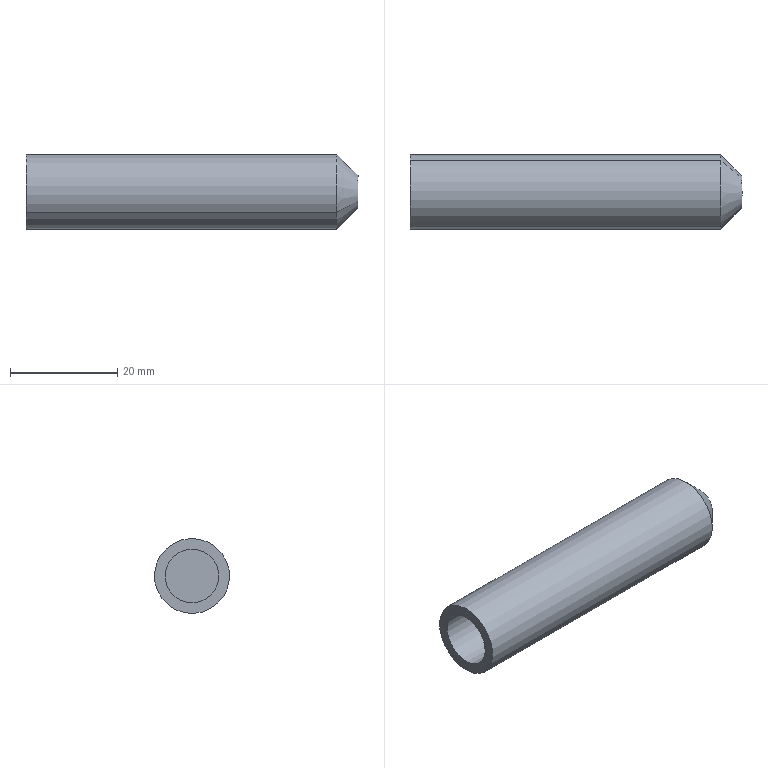Component | SolidWorks | HZ022-A001-E006-1 | 1 solid | 9 faces | box 62 x 14 x 14 mm | volume 7485 mm3 | cylinder 4 | plane 3 | cone 2 | commonest cylinder face diameters 10.02 x2 14 x2 | material S45C
build123d program:
from build123d import *

# Parameters (mm, degrees)
SKETCH1_2_R             = 7
BOSS_EXTRUDE1_DEPTH     = 62
CHAMFER1_SIZE           = 4
CUT_EXTRUDE1_DEPTH      = 22.5
CUT_EXTRUDE1_DEPTH_BACK = 22.5
SKETCH1_R               = 5.01


with BuildPart() as part:
    # Sketch1_2 → Boss-Extrude1 (new body)
    with BuildSketch(Plane(origin=(0, 0, 0), x_dir=(1, 0, 0), z_dir=(0, 1, 0))):
        with Locations(Location((0, 0, 0), (0, 0, 270))):
            Circle(SKETCH1_2_R)
    extrude(amount=BOSS_EXTRUDE1_DEPTH)

    # Chamfer1
    chamfer1_edges = [part.edges().sort_by_distance(p)[0] for p in [
        (0, 62, -7),
    ]]
    chamfer(chamfer1_edges, length=CHAMFER1_SIZE)

    # Sketch1 → Cut-Extrude1 (cut, two sides: drawn at the far end of the back side and taken through both)
    with BuildSketch(Plane(origin=(0, 0, 0), x_dir=(1, 0, 0), z_dir=(0, 1, 0)).offset(-CUT_EXTRUDE1_DEPTH_BACK)):
        with Locations(Location((0, 0, 0), (0, 0, 90))):
            Circle(SKETCH1_R)
    extrude(amount=CUT_EXTRUDE1_DEPTH + CUT_EXTRUDE1_DEPTH_BACK, mode=Mode.SUBTRACT)


solid = part.part

# Placed as in the assembly
solid = solid.moved(Location((-64.556, 126.652, 927), (0, 0, -90)))
STEP:
#1=COLOUR_RGB('',0.7922,0.8196,0.9333);
#2=FILL_AREA_STYLE_COLOUR('',#1);
#3=FILL_AREA_STYLE('',(#2));
#4=SURFACE_STYLE_FILL_AREA(#3);
#5=SURFACE_SIDE_STYLE('',(#4));
#6=SURFACE_STYLE_USAGE(.BOTH.,#5);
#7=PRESENTATION_STYLE_ASSIGNMENT((#6));
#8=CARTESIAN_POINT('',(-1.656,5.153,36.602));
#9=VERTEX_POINT('',#8);
#10=CARTESIAN_POINT('',(-1.656,4.82,36.39));
#11=VERTEX_POINT('',#10);
#12=CARTESIAN_POINT('',(-1.656,4.986,36.496));
#13=DIRECTION('',(1.,0.,-0.));
#14=DIRECTION('',(-0.,-0.8435,-0.5371));
#15=AXIS2_PLACEMENT_3D('',#12,#13,#14);
#16=CIRCLE('',#15,0.1972);
#17=EDGE_CURVE('',#9,#11,#16,.T.);
#18=ORIENTED_EDGE('',*,*,#17,.T.);
#19=CARTESIAN_POINT('',(-2.542,4.82,36.39));
#20=VERTEX_POINT('',#19);
#21=CARTESIAN_POINT('',(-1.656,4.82,36.39));
#22=DIRECTION('',(-1.,-0.,0.));
#23=VECTOR('',#22,39.37);
#24=LINE('',#21,#23);
#25=EDGE_CURVE('',#11,#20,#24,.T.);
#26=ORIENTED_EDGE('',*,*,#25,.T.);
#27=CARTESIAN_POINT('',(-2.542,5.153,36.602));
#28=VERTEX_POINT('',#27);
#29=CARTESIAN_POINT('',(-2.542,4.986,36.496));
#30=DIRECTION('',(-1.,-0.,0.));
#31=DIRECTION('',(-0.,-0.8435,-0.5371));
#32=AXIS2_PLACEMENT_3D('',#29,#30,#31);
#33=CIRCLE('',#32,0.1972);
#34=EDGE_CURVE('',#20,#28,#33,.T.);
#35=ORIENTED_EDGE('',*,*,#34,.T.);
#36=CARTESIAN_POINT('',(-1.656,5.153,36.602));
#37=DIRECTION('',(-1.,-0.,0.));
#38=VECTOR('',#37,39.37);
#39=LINE('',#36,#38);
#40=EDGE_CURVE('',#9,#28,#39,.T.);
#41=ORIENTED_EDGE('',*,*,#40,.F.);
#42=EDGE_LOOP('',(#18,#26,#35,#41));
#43=FACE_OUTER_BOUND('',#42,.T.);
#44=CARTESIAN_POINT('',(-1.656,4.986,36.496));
#45=DIRECTION('',(-1.,-0.,0.));
#46=DIRECTION('',(0.,0.8435,0.5371));
#47=AXIS2_PLACEMENT_3D('',#44,#45,#46);
#48=CYLINDRICAL_SURFACE('',#47,0.1972);
#49=ADVANCED_FACE('',(#43),#48,.F.);
#50=CARTESIAN_POINT('',(-0.1006,4.887,36.433));
#51=VERTEX_POINT('',#50);
#52=CARTESIAN_POINT('',(-0.1006,5.086,36.559));
#53=VERTEX_POINT('',#52);
#54=CARTESIAN_POINT('',(-0.1006,4.986,36.496));
#55=DIRECTION('',(1.,0.,-0.));
#56=DIRECTION('',(-0.,-0.8435,-0.5371));
#57=AXIS2_PLACEMENT_3D('',#54,#55,#56);
#58=CIRCLE('',#57,0.1181);
#59=EDGE_CURVE('',#51,#53,#58,.T.);
#60=ORIENTED_EDGE('',*,*,#59,.F.);
#61=CARTESIAN_POINT('',(-0.2581,4.754,36.348));
#62=VERTEX_POINT('',#61);
#63=CARTESIAN_POINT('',(-0.1006,4.887,36.433));
#64=DIRECTION('',(-0.7071,-0.5965,-0.3798));
#65=VECTOR('',#64,39.37);
#66=LINE('',#63,#65);
#67=EDGE_CURVE('',#51,#62,#66,.T.);
#68=ORIENTED_EDGE('',*,*,#67,.T.);
#69=CARTESIAN_POINT('',(-0.2581,5.219,36.644));
#70=VERTEX_POINT('',#69);
#71=CARTESIAN_POINT('',(-0.2581,4.986,36.496));
#72=DIRECTION('',(-1.,-0.,0.));
#73=DIRECTION('',(-0.,-0.8435,-0.5371));
#74=AXIS2_PLACEMENT_3D('',#71,#72,#73);
#75=CIRCLE('',#74,0.2756);
#76=EDGE_CURVE('',#70,#62,#75,.T.);
#77=ORIENTED_EDGE('',*,*,#76,.F.);
#78=CARTESIAN_POINT('',(-0.1006,5.086,36.559));
#79=DIRECTION('',(-0.7071,0.5965,0.3798));
#80=VECTOR('',#79,39.37);
#81=LINE('',#78,#80);
#82=EDGE_CURVE('',#53,#70,#81,.T.);
#83=ORIENTED_EDGE('',*,*,#82,.F.);
#84=EDGE_LOOP('',(#60,#68,#77,#83));
#85=FACE_OUTER_BOUND('',#84,.T.);
#86=CARTESIAN_POINT('',(-0.1006,4.986,36.496));
#87=DIRECTION('',(-1.,-0.,0.));
#88=DIRECTION('',(0.,0.8435,0.5371));
#89=AXIS2_PLACEMENT_3D('',#86,#87,#88);
#90=CONICAL_SURFACE('',#89,0.1181,0.7854);
#91=ADVANCED_FACE('',(#85),#90,.T.);
#92=ORIENTED_EDGE('',*,*,#76,.T.);
#93=CARTESIAN_POINT('',(-2.542,4.754,36.348));
#94=VERTEX_POINT('',#93);
#95=CARTESIAN_POINT('',(-0.1006,4.754,36.348));
#96=DIRECTION('',(-1.,-0.,0.));
#97=VECTOR('',#96,39.37);
#98=LINE('',#95,#97);
#99=EDGE_CURVE('',#62,#94,#98,.T.);
#100=ORIENTED_EDGE('',*,*,#99,.T.);
#101=CARTESIAN_POINT('',(-2.542,5.219,36.644));
#102=VERTEX_POINT('',#101);
#103=CARTESIAN_POINT('',(-2.542,4.986,36.496));
#104=DIRECTION('',(1.,0.,-0.));
#105=DIRECTION('',(-0.,-0.8435,-0.5371));
#106=AXIS2_PLACEMENT_3D('',#103,#104,#105);
#107=CIRCLE('',#106,0.2756);
#108=EDGE_CURVE('',#94,#102,#107,.T.);
#109=ORIENTED_EDGE('',*,*,#108,.T.);
#110=CARTESIAN_POINT('',(-0.1006,5.219,36.644));
#111=DIRECTION('',(-1.,-0.,0.));
#112=VECTOR('',#111,39.37);
#113=LINE('',#110,#112);
#114=EDGE_CURVE('',#70,#102,#113,.T.);
#115=ORIENTED_EDGE('',*,*,#114,.F.);
#116=EDGE_LOOP('',(#92,#100,#109,#115));
#117=FACE_OUTER_BOUND('',#116,.T.);
#118=CARTESIAN_POINT('',(-0.1006,4.986,36.496));
#119=DIRECTION('',(-1.,-0.,0.));
#120=DIRECTION('',(0.,0.8435,0.5371));
#121=AXIS2_PLACEMENT_3D('',#118,#119,#120);
#122=CYLINDRICAL_SURFACE('',#121,0.2756);
#123=ADVANCED_FACE('',(#117),#122,.T.);
#124=ORIENTED_EDGE('',*,*,#99,.F.);
#125=CARTESIAN_POINT('',(-0.2581,4.986,36.496));
#126=DIRECTION('',(-1.,-0.,0.));
#127=DIRECTION('',(-0.,-0.8435,-0.5371));
#128=AXIS2_PLACEMENT_3D('',#125,#126,#127);
#129=CIRCLE('',#128,0.2756);
#130=EDGE_CURVE('',#62,#70,#129,.T.);
#131=ORIENTED_EDGE('',*,*,#130,.T.);
#132=ORIENTED_EDGE('',*,*,#114,.T.);
#133=CARTESIAN_POINT('',(-2.542,4.986,36.496));
#134=DIRECTION('',(1.,0.,-0.));
#135=DIRECTION('',(-0.,-0.8435,-0.5371));
#136=AXIS2_PLACEMENT_3D('',#133,#134,#135);
#137=CIRCLE('',#136,0.2756);
#138=EDGE_CURVE('',#102,#94,#137,.T.);
#139=ORIENTED_EDGE('',*,*,#138,.T.);
#140=EDGE_LOOP('',(#124,#131,#132,#139));
#141=FACE_OUTER_BOUND('',#140,.T.);
#142=CARTESIAN_POINT('',(-0.1006,4.986,36.496));
#143=DIRECTION('',(-1.,-0.,0.));
#144=DIRECTION('',(0.,0.8435,0.5371));
#145=AXIS2_PLACEMENT_3D('',#142,#143,#144);
#146=CYLINDRICAL_SURFACE('',#145,0.2756);
#147=ADVANCED_FACE('',(#141),#146,.T.);
#148=CARTESIAN_POINT('',(-0.1006,4.986,36.496));
#149=DIRECTION('',(1.,0.,-0.));
#150=DIRECTION('',(-0.,-0.8435,-0.5371));
#151=AXIS2_PLACEMENT_3D('',#148,#149,#150);
#152=CIRCLE('',#151,0.1181);
#153=EDGE_CURVE('',#53,#51,#152,.T.);
#154=ORIENTED_EDGE('',*,*,#153,.T.);
#155=ORIENTED_EDGE('',*,*,#59,.T.);
#156=EDGE_LOOP('',(#154,#155));
#157=FACE_OUTER_BOUND('',#156,.T.);
#158=CARTESIAN_POINT('',(-0.1006,4.986,36.496));
#159=DIRECTION('',(1.,0.,-0.));
#160=DIRECTION('',(-0.,-0.8435,-0.5371));
#161=AXIS2_PLACEMENT_3D('',#158,#159,#160);
#162=PLANE('',#161);
#163=ADVANCED_FACE('',(#157),#162,.T.);
#164=CARTESIAN_POINT('',(-2.542,4.986,36.496));
#165=DIRECTION('',(-1.,-0.,0.));
#166=DIRECTION('',(-0.,-0.8435,-0.5371));
#167=AXIS2_PLACEMENT_3D('',#164,#165,#166);
#168=CIRCLE('',#167,0.1972);
#169=EDGE_CURVE('',#28,#20,#168,.T.);
#170=ORIENTED_EDGE('',*,*,#169,.F.);
#171=ORIENTED_EDGE('',*,*,#34,.F.);
#172=EDGE_LOOP('',(#170,#171));
#173=FACE_BOUND('',#172,.T.);
#174=ORIENTED_EDGE('',*,*,#138,.F.);
#175=ORIENTED_EDGE('',*,*,#108,.F.);
#176=EDGE_LOOP('',(#174,#175));
#177=FACE_OUTER_BOUND('',#176,.T.);
#178=CARTESIAN_POINT('',(-2.542,4.986,36.496));
#179=DIRECTION('',(1.,0.,-0.));
#180=DIRECTION('',(-0.,-0.8435,-0.5371));
#181=AXIS2_PLACEMENT_3D('',#178,#179,#180);
#182=PLANE('',#181);
#183=ADVANCED_FACE('',(#173,#177),#182,.F.);
#184=ORIENTED_EDGE('',*,*,#67,.F.);
#185=ORIENTED_EDGE('',*,*,#153,.F.);
#186=ORIENTED_EDGE('',*,*,#82,.T.);
#187=ORIENTED_EDGE('',*,*,#130,.F.);
#188=EDGE_LOOP('',(#184,#185,#186,#187));
#189=FACE_OUTER_BOUND('',#188,.T.);
#190=CARTESIAN_POINT('',(-0.1006,4.986,36.496));
#191=DIRECTION('',(-1.,-0.,0.));
#192=DIRECTION('',(0.,0.8435,0.5371));
#193=AXIS2_PLACEMENT_3D('',#190,#191,#192);
#194=CONICAL_SURFACE('',#193,0.1181,0.7854);
#195=ADVANCED_FACE('',(#189),#194,.T.);
#196=ORIENTED_EDGE('',*,*,#25,.F.);
#197=CARTESIAN_POINT('',(-1.656,4.986,36.496));
#198=DIRECTION('',(1.,0.,-0.));
#199=DIRECTION('',(-0.,-0.8435,-0.5371));
#200=AXIS2_PLACEMENT_3D('',#197,#198,#199);
#201=CIRCLE('',#200,0.1972);
#202=EDGE_CURVE('',#11,#9,#201,.T.);
#203=ORIENTED_EDGE('',*,*,#202,.T.);
#204=ORIENTED_EDGE('',*,*,#40,.T.);
#205=ORIENTED_EDGE('',*,*,#169,.T.);
#206=EDGE_LOOP('',(#196,#203,#204,#205));
#207=FACE_OUTER_BOUND('',#206,.T.);
#208=CARTESIAN_POINT('',(-1.656,4.986,36.496));
#209=DIRECTION('',(-1.,-0.,0.));
#210=DIRECTION('',(0.,0.8435,0.5371));
#211=AXIS2_PLACEMENT_3D('',#208,#209,#210);
#212=CYLINDRICAL_SURFACE('',#211,0.1972);
#213=ADVANCED_FACE('',(#207),#212,.F.);
#214=ORIENTED_EDGE('',*,*,#17,.F.);
#215=ORIENTED_EDGE('',*,*,#202,.F.);
#216=EDGE_LOOP('',(#214,#215));
#217=FACE_OUTER_BOUND('',#216,.T.);
#218=CARTESIAN_POINT('',(-1.656,4.986,36.496));
#219=DIRECTION('',(1.,0.,-0.));
#220=DIRECTION('',(-0.,-0.8435,-0.5371));
#221=AXIS2_PLACEMENT_3D('',#218,#219,#220);
#222=PLANE('',#221);
#223=ADVANCED_FACE('',(#217),#222,.F.);
#224=CLOSED_SHELL('',(#49,#91,#123,#147,#163,#183,#195,#213,#223));
#225=MANIFOLD_SOLID_BREP('',#224);
#226=STYLED_ITEM('',(#7),#225);
#227=(LENGTH_UNIT()NAMED_UNIT(*)SI_UNIT($,.METRE.));
#228=LENGTH_MEASURE_WITH_UNIT(LENGTH_MEASURE(0.0254),#227);
#229=DIMENSIONAL_EXPONENTS(1.,0.,0.,0.,0.,0.,0.);
#230=(CONVERSION_BASED_UNIT('',#228)LENGTH_UNIT()NAMED_UNIT(#229));
#231=UNCERTAINTY_MEASURE_WITH_UNIT(LENGTH_MEASURE(0.00001),#230,'','');
#232=(NAMED_UNIT(*)PLANE_ANGLE_UNIT()SI_UNIT($,.RADIAN.));
#233=(NAMED_UNIT(*)SI_UNIT($,.STERADIAN.)SOLID_ANGLE_UNIT());
#234=(GEOMETRIC_REPRESENTATION_CONTEXT(3)GLOBAL_UNCERTAINTY_ASSIGNED_CONTEXT((#231))GLOBAL_UNIT_ASSIGNED_CONTEXT((#230,#232,#233))REPRESENTATION_CONTEXT('',''));
#235=MECHANICAL_DESIGN_GEOMETRIC_PRESENTATION_REPRESENTATION('',(#226),#234);
#236=PRESENTATION_LAYER_ASSIGNMENT('','',(#226));
#237=CARTESIAN_POINT('',(0.,0.,0.));
#238=DIRECTION('',(0.,0.,1.));
#239=DIRECTION('',(1.,0.,0.));
#240=AXIS2_PLACEMENT_3D('',#237,#238,#239);
#241=(LENGTH_UNIT()NAMED_UNIT(*)SI_UNIT($,.METRE.));
#242=LENGTH_MEASURE_WITH_UNIT(LENGTH_MEASURE(0.0254),#241);
#243=DIMENSIONAL_EXPONENTS(1.,0.,0.,0.,0.,0.,0.);
#244=(CONVERSION_BASED_UNIT('',#242)LENGTH_UNIT()NAMED_UNIT(#243));
#245=UNCERTAINTY_MEASURE_WITH_UNIT(LENGTH_MEASURE(0.00001),#244,'','');
#246=(NAMED_UNIT(*)PLANE_ANGLE_UNIT()SI_UNIT($,.RADIAN.));
#247=(NAMED_UNIT(*)SI_UNIT($,.STERADIAN.)SOLID_ANGLE_UNIT());
#248=(GEOMETRIC_REPRESENTATION_CONTEXT(3)GLOBAL_UNCERTAINTY_ASSIGNED_CONTEXT((#245))GLOBAL_UNIT_ASSIGNED_CONTEXT((#244,#246,#247))REPRESENTATION_CONTEXT('',''));
#249=ADVANCED_BREP_SHAPE_REPRESENTATION('',(#225,#240),#248);